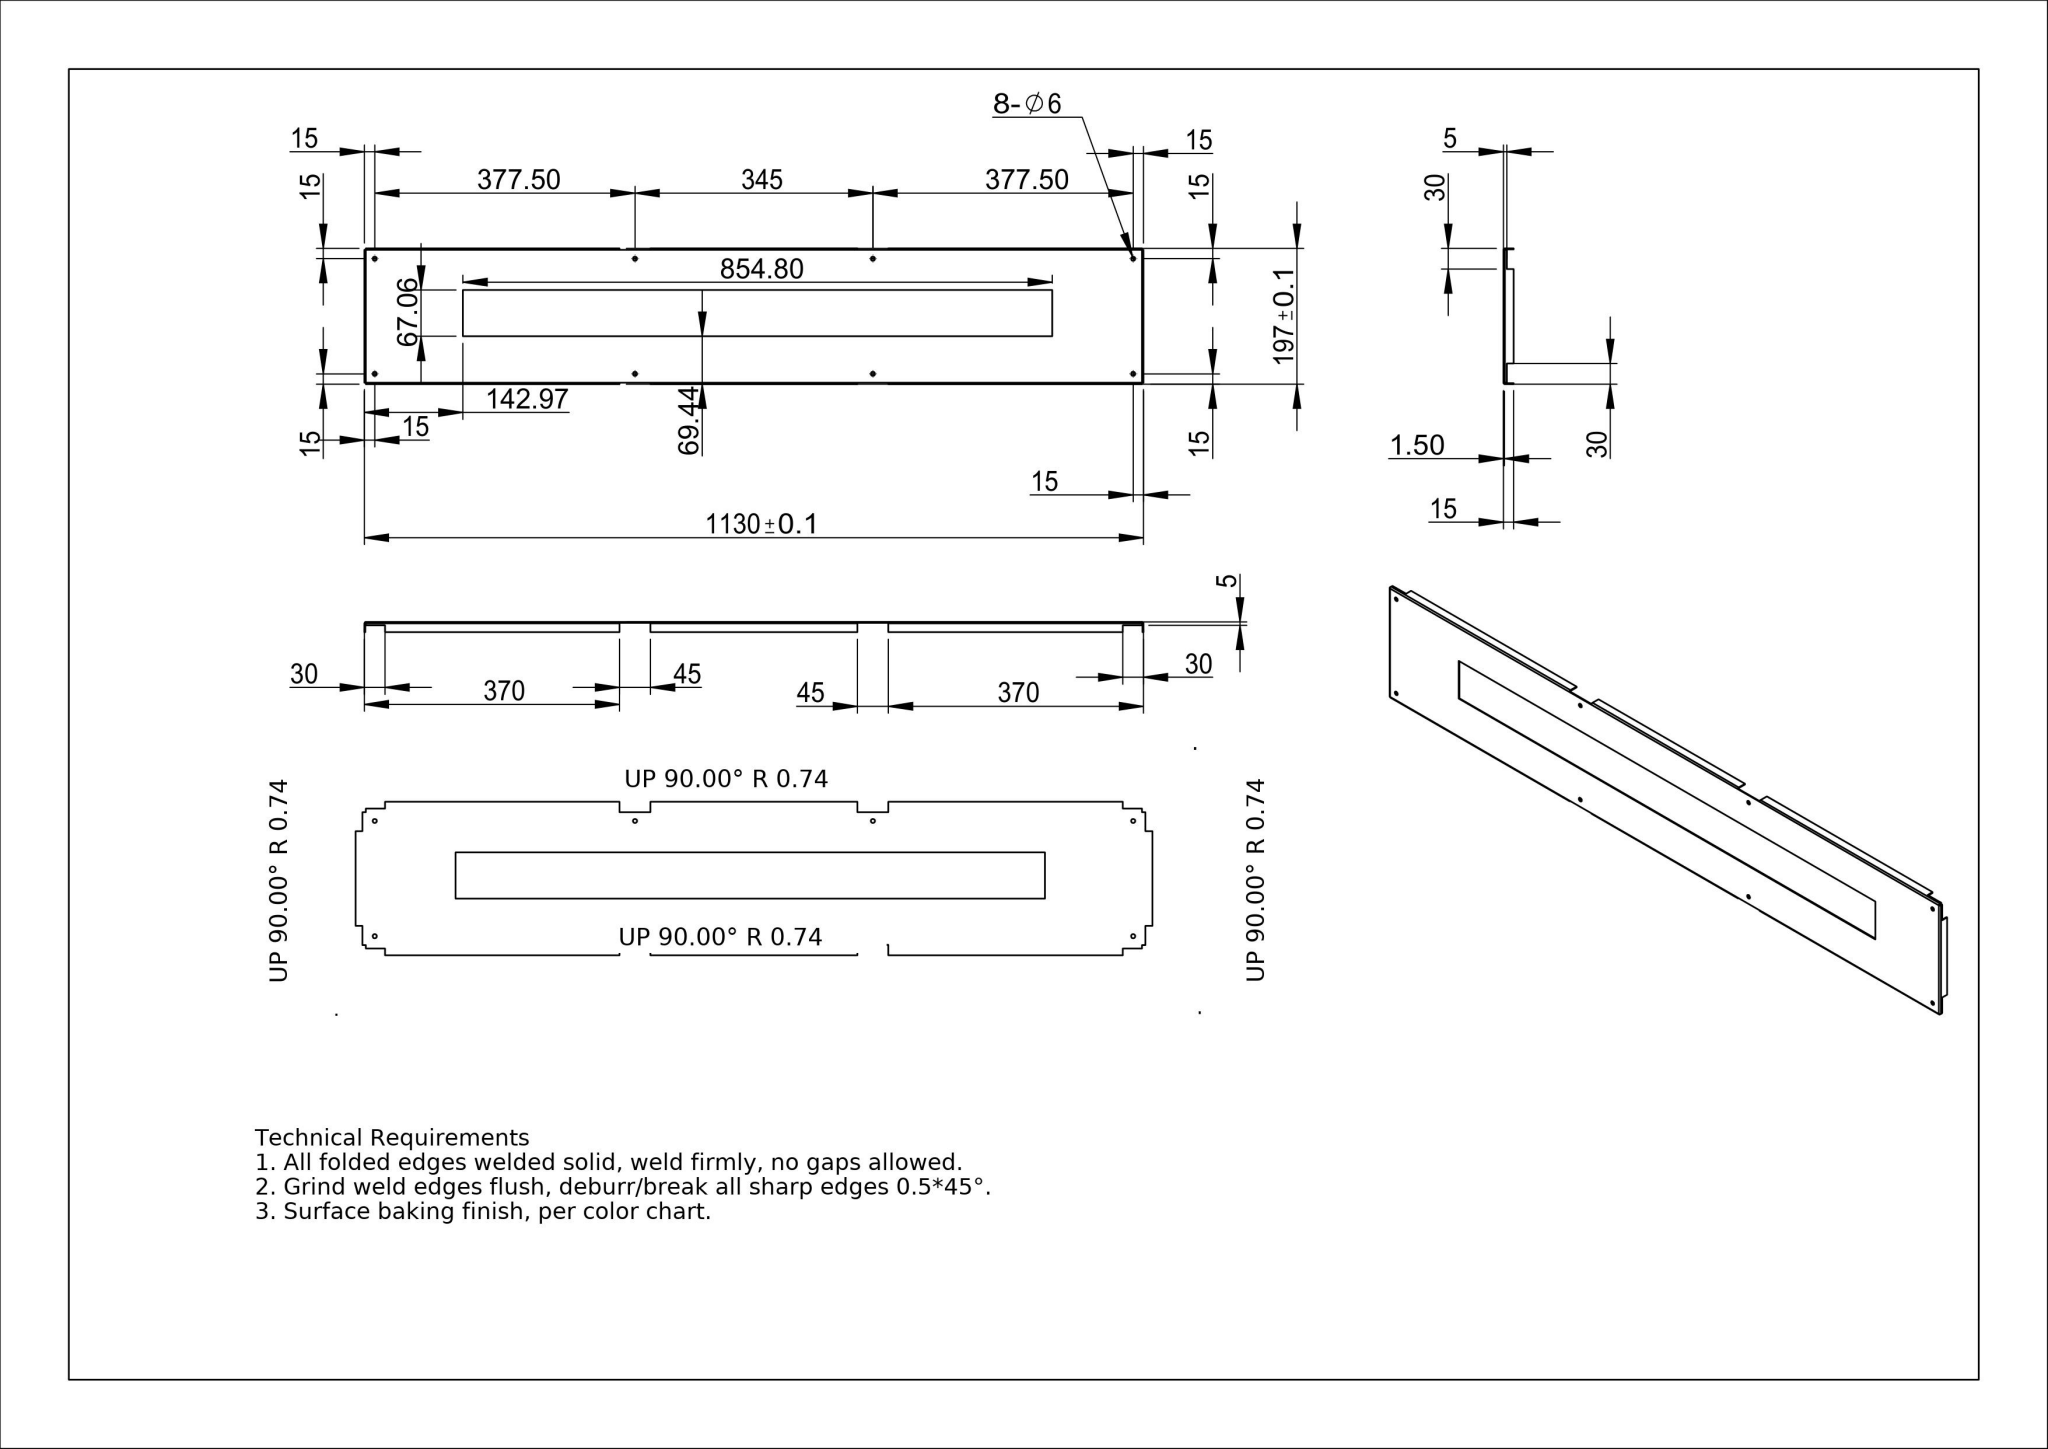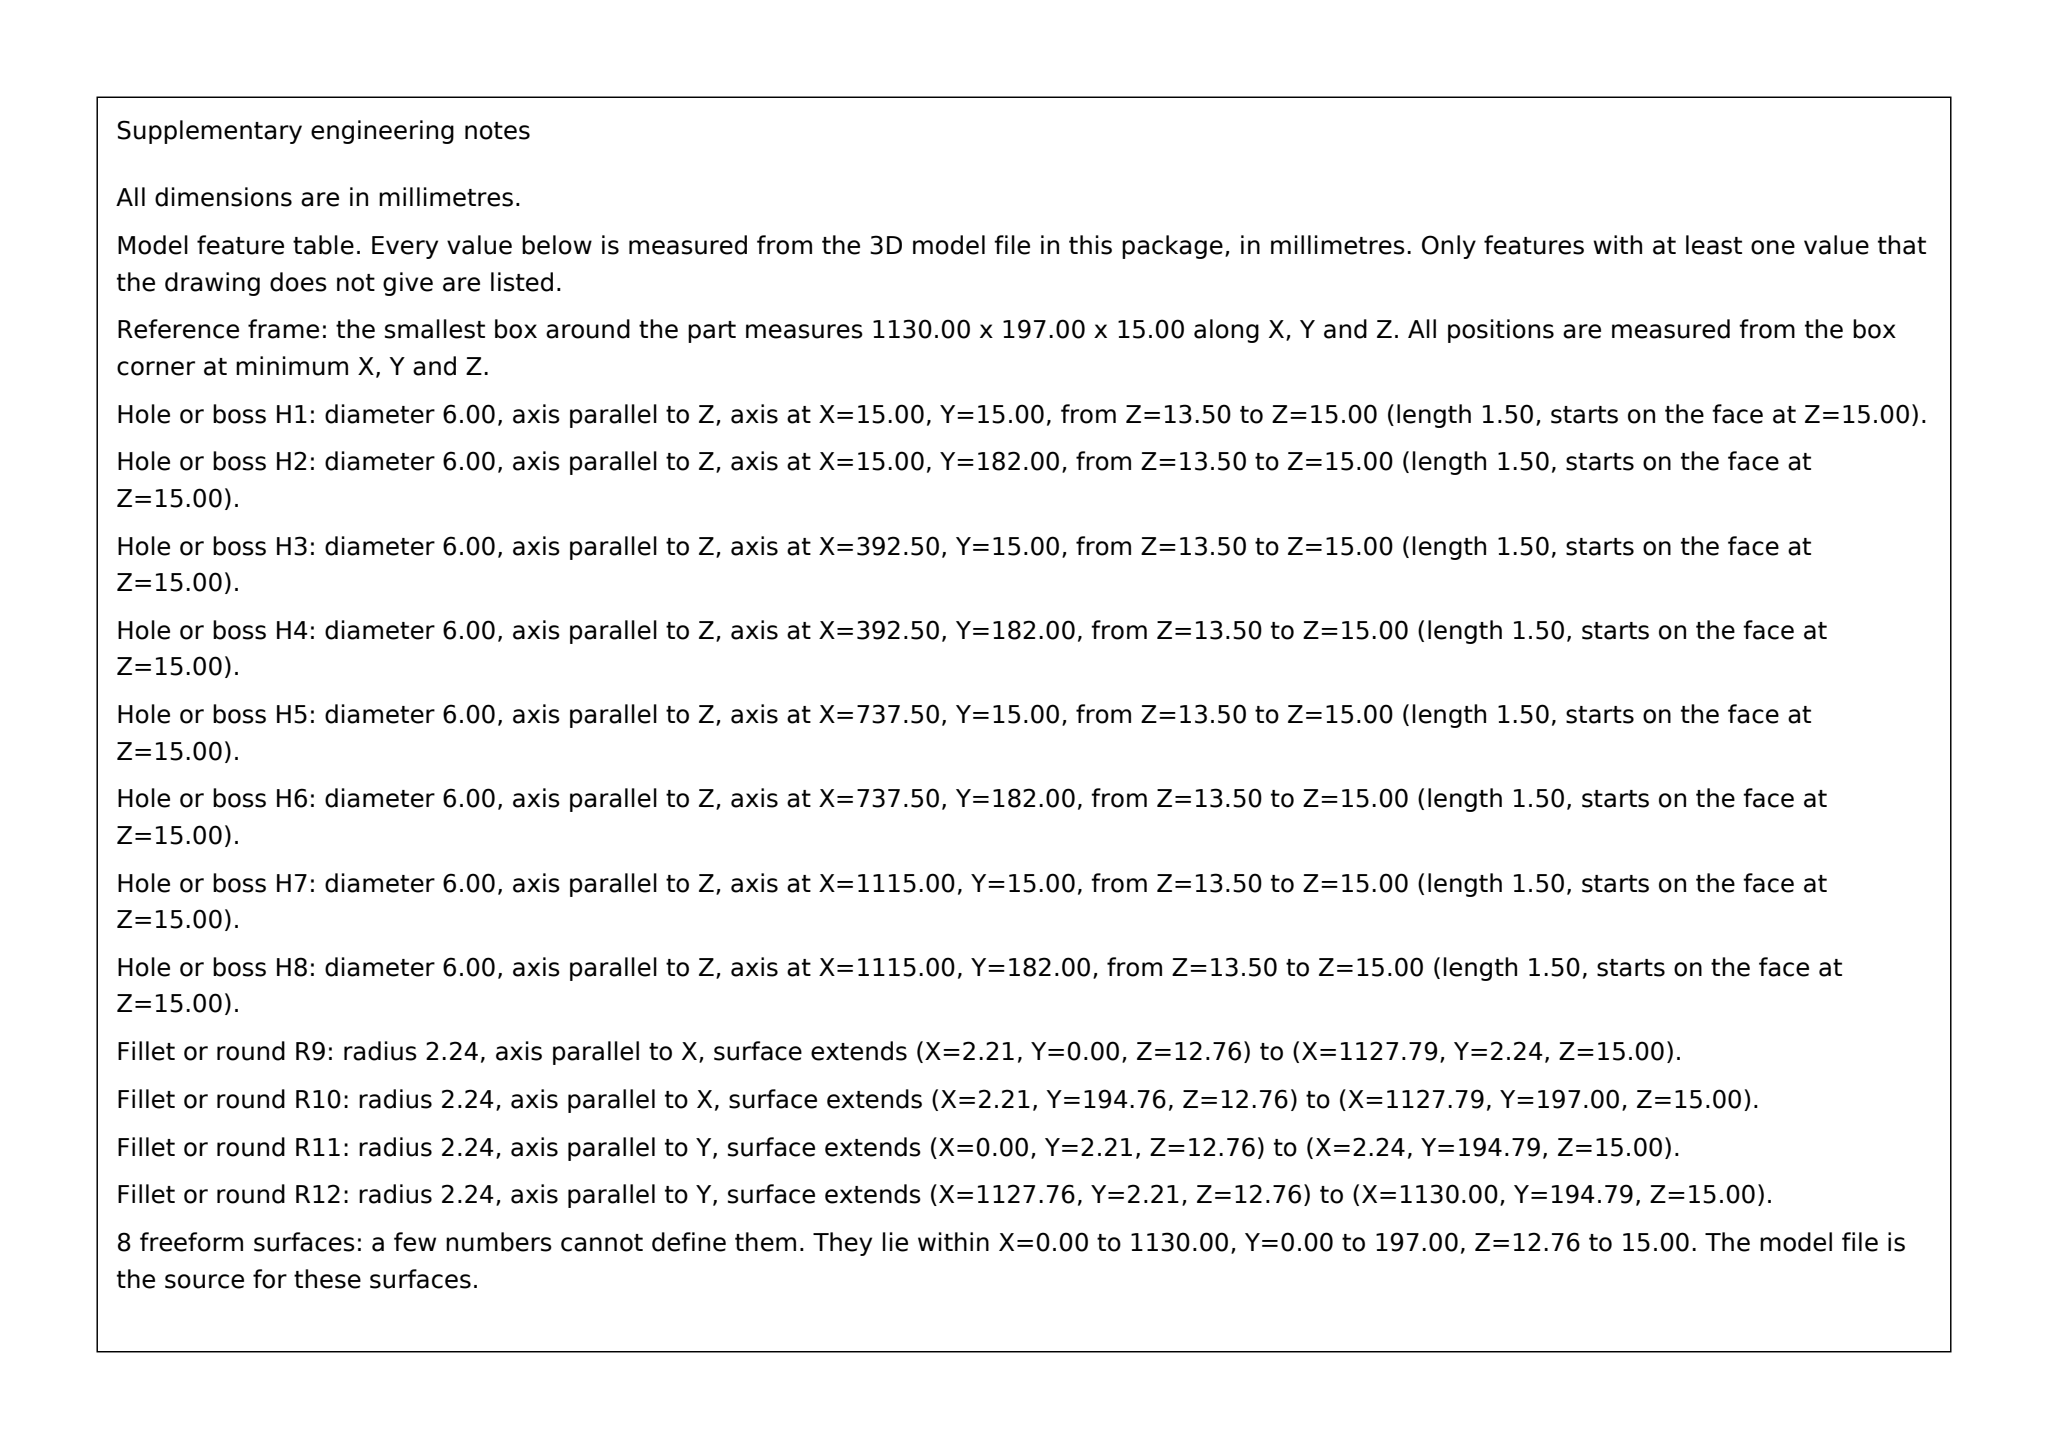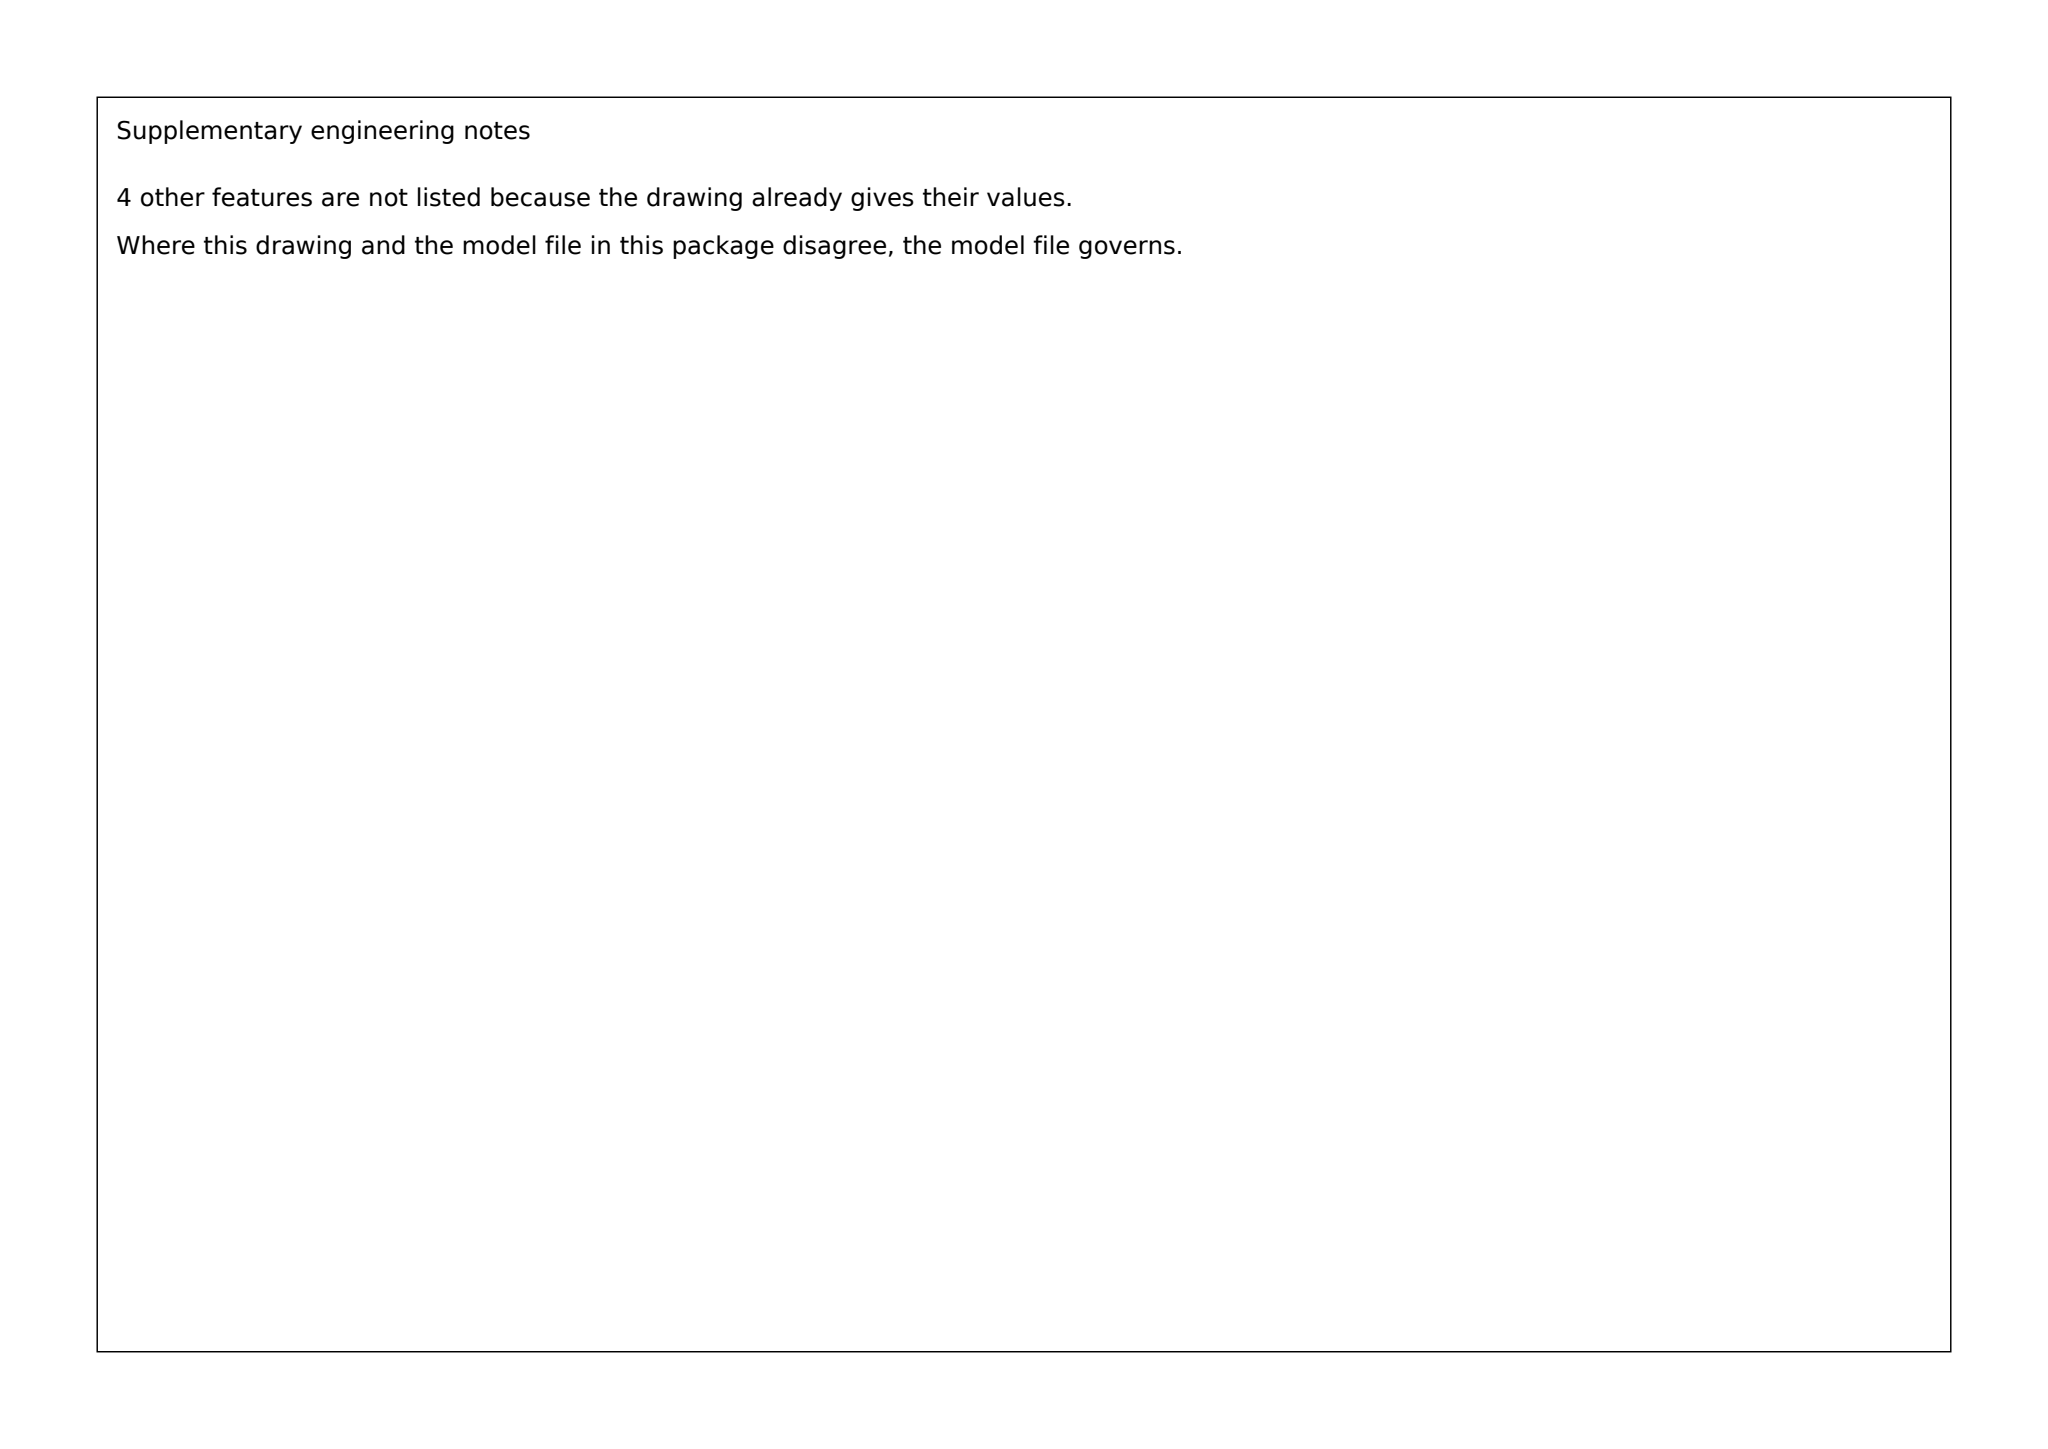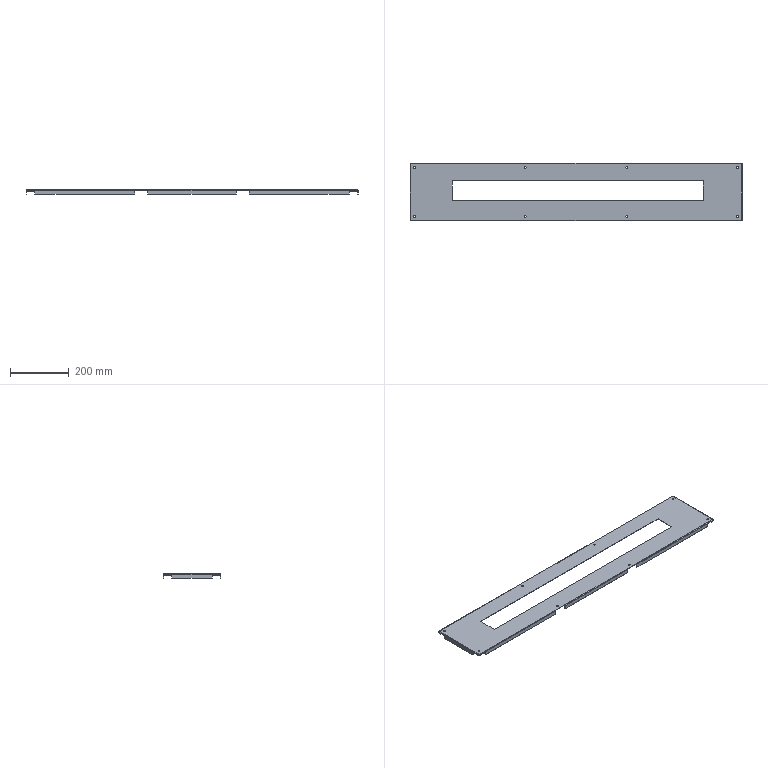Part | SolidWorks | mm | 1 solid | 114 faces | box 1130 x 197 x 15 mm | volume 291012 mm3 | plane 74 | cylinder 32 | spline 8 | commonest cylinder face diameters 6 x16 4.473 x8 1.473 x8